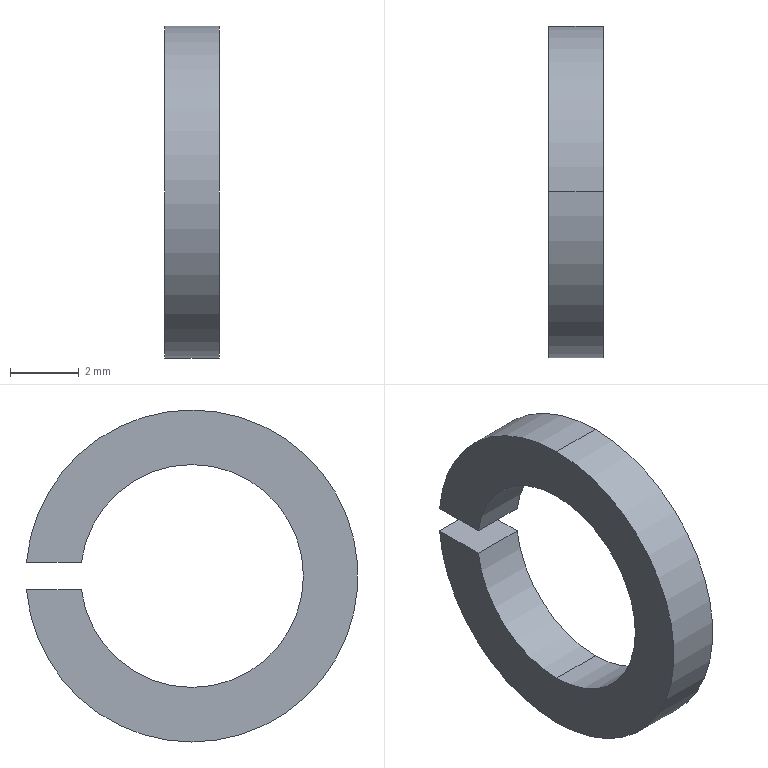Component | SolidWorks | GB_T93-1987StandardTypeSpringWasher(Assembly)6x1.6-1 | 1 solid | 10 faces | box 1.6 x 9.67 x 9.68 mm | volume 63 mm3 | cylinder 6 | plane 4 | commonest cylinder face diameters 6.5 x3 9.684 x3
build123d program:
from build123d import *

# Parameters (mm, degrees)
EXTRUDE1_DEPTH = 1.6


with BuildPart() as part:
    # Sketch1 → Extrude1 (new body)
    with BuildSketch(Plane.XY):
        with BuildLine():
            Line((-0.4, 4.825), (-0.4, 3.225))
            ThreePointArc((-0.4, 3.225), (0, -3.25), (0.4, 3.225))
            Line((0.4, 3.225), (0.4, 4.825))
            ThreePointArc((0.4, 4.825), (0, -4.842), (-0.4, 4.825))
        make_face()
    extrude(amount=EXTRUDE1_DEPTH)


solid = part.part

# Placed as in the assembly
solid = solid.moved(Location((-514.8, 30, 325), (0, 90, 0)))
STEP:
#1=CARTESIAN_POINT('',(-20.205,1.181,12.667));
#2=VERTEX_POINT('',#1);
#3=CARTESIAN_POINT('',(-20.205,1.181,12.923));
#4=VERTEX_POINT('',#3);
#5=CARTESIAN_POINT('',(-20.205,1.181,12.795));
#6=DIRECTION('',(-1.,0.,0.));
#7=DIRECTION('',(0.,0.,-1.));
#8=AXIS2_PLACEMENT_3D('',#5,#6,#7);
#9=CIRCLE('',#8,0.128);
#10=EDGE_CURVE('',#2,#4,#9,.T.);
#11=ORIENTED_EDGE('',*,*,#10,.F.);
#12=CARTESIAN_POINT('',(-20.268,1.181,12.667));
#13=VERTEX_POINT('',#12);
#14=CARTESIAN_POINT('',(-20.205,1.181,12.667));
#15=DIRECTION('',(-1.,0.,0.));
#16=VECTOR('',#15,39.37);
#17=LINE('',#14,#16);
#18=EDGE_CURVE('',#2,#13,#17,.T.);
#19=ORIENTED_EDGE('',*,*,#18,.T.);
#20=CARTESIAN_POINT('',(-20.268,1.181,12.923));
#21=VERTEX_POINT('',#20);
#22=CARTESIAN_POINT('',(-20.268,1.181,12.795));
#23=DIRECTION('',(-1.,0.,0.));
#24=DIRECTION('',(0.,0.,-1.));
#25=AXIS2_PLACEMENT_3D('',#22,#23,#24);
#26=CIRCLE('',#25,0.128);
#27=EDGE_CURVE('',#13,#21,#26,.T.);
#28=ORIENTED_EDGE('',*,*,#27,.T.);
#29=CARTESIAN_POINT('',(-20.205,1.181,12.923));
#30=DIRECTION('',(-1.,0.,0.));
#31=VECTOR('',#30,39.37);
#32=LINE('',#29,#31);
#33=EDGE_CURVE('',#4,#21,#32,.T.);
#34=ORIENTED_EDGE('',*,*,#33,.F.);
#35=EDGE_LOOP('',(#11,#19,#28,#34));
#36=FACE_OUTER_BOUND('',#35,.T.);
#37=CARTESIAN_POINT('',(-20.205,1.181,12.795));
#38=DIRECTION('',(-1.,0.,0.));
#39=DIRECTION('',(0.,0.,1.));
#40=AXIS2_PLACEMENT_3D('',#37,#38,#39);
#41=CYLINDRICAL_SURFACE('',#40,0.128);
#42=ADVANCED_FACE('',(#36),#41,.F.);
#43=CARTESIAN_POINT('',(-20.205,1.308,12.811));
#44=VERTEX_POINT('',#43);
#45=CARTESIAN_POINT('',(-20.205,1.181,12.795));
#46=DIRECTION('',(-1.,0.,0.));
#47=DIRECTION('',(0.,0.,-1.));
#48=AXIS2_PLACEMENT_3D('',#45,#46,#47);
#49=CIRCLE('',#48,0.128);
#50=EDGE_CURVE('',#4,#44,#49,.T.);
#51=ORIENTED_EDGE('',*,*,#50,.F.);
#52=ORIENTED_EDGE('',*,*,#33,.T.);
#53=CARTESIAN_POINT('',(-20.268,1.308,12.811));
#54=VERTEX_POINT('',#53);
#55=CARTESIAN_POINT('',(-20.268,1.181,12.795));
#56=DIRECTION('',(-1.,0.,0.));
#57=DIRECTION('',(0.,0.,-1.));
#58=AXIS2_PLACEMENT_3D('',#55,#56,#57);
#59=CIRCLE('',#58,0.128);
#60=EDGE_CURVE('',#21,#54,#59,.T.);
#61=ORIENTED_EDGE('',*,*,#60,.T.);
#62=CARTESIAN_POINT('',(-20.205,1.308,12.811));
#63=DIRECTION('',(-1.,0.,0.));
#64=VECTOR('',#63,39.37);
#65=LINE('',#62,#64);
#66=EDGE_CURVE('',#44,#54,#65,.T.);
#67=ORIENTED_EDGE('',*,*,#66,.F.);
#68=EDGE_LOOP('',(#51,#52,#61,#67));
#69=FACE_OUTER_BOUND('',#68,.T.);
#70=CARTESIAN_POINT('',(-20.205,1.181,12.795));
#71=DIRECTION('',(-1.,0.,0.));
#72=DIRECTION('',(0.,0.,1.));
#73=AXIS2_PLACEMENT_3D('',#70,#71,#72);
#74=CYLINDRICAL_SURFACE('',#73,0.128);
#75=ADVANCED_FACE('',(#69),#74,.F.);
#76=CARTESIAN_POINT('',(-20.205,1.181,12.605));
#77=VERTEX_POINT('',#76);
#78=CARTESIAN_POINT('',(-20.205,1.371,12.78));
#79=VERTEX_POINT('',#78);
#80=CARTESIAN_POINT('',(-20.205,1.181,12.795));
#81=DIRECTION('',(1.,0.,0.));
#82=DIRECTION('',(0.,0.,-1.));
#83=AXIS2_PLACEMENT_3D('',#80,#81,#82);
#84=CIRCLE('',#83,0.1906);
#85=EDGE_CURVE('',#77,#79,#84,.T.);
#86=ORIENTED_EDGE('',*,*,#85,.F.);
#87=CARTESIAN_POINT('',(-20.268,1.181,12.605));
#88=VERTEX_POINT('',#87);
#89=CARTESIAN_POINT('',(-20.205,1.181,12.605));
#90=DIRECTION('',(-1.,0.,0.));
#91=VECTOR('',#90,39.37);
#92=LINE('',#89,#91);
#93=EDGE_CURVE('',#77,#88,#92,.T.);
#94=ORIENTED_EDGE('',*,*,#93,.T.);
#95=CARTESIAN_POINT('',(-20.268,1.371,12.78));
#96=VERTEX_POINT('',#95);
#97=CARTESIAN_POINT('',(-20.268,1.181,12.795));
#98=DIRECTION('',(1.,0.,0.));
#99=DIRECTION('',(0.,0.,-1.));
#100=AXIS2_PLACEMENT_3D('',#97,#98,#99);
#101=CIRCLE('',#100,0.1906);
#102=EDGE_CURVE('',#88,#96,#101,.T.);
#103=ORIENTED_EDGE('',*,*,#102,.T.);
#104=CARTESIAN_POINT('',(-20.205,1.371,12.78));
#105=DIRECTION('',(-1.,0.,0.));
#106=VECTOR('',#105,39.37);
#107=LINE('',#104,#106);
#108=EDGE_CURVE('',#79,#96,#107,.T.);
#109=ORIENTED_EDGE('',*,*,#108,.F.);
#110=EDGE_LOOP('',(#86,#94,#103,#109));
#111=FACE_OUTER_BOUND('',#110,.T.);
#112=CARTESIAN_POINT('',(-20.205,1.181,12.795));
#113=DIRECTION('',(-1.,0.,0.));
#114=DIRECTION('',(0.,0.,1.));
#115=AXIS2_PLACEMENT_3D('',#112,#113,#114);
#116=CYLINDRICAL_SURFACE('',#115,0.1906);
#117=ADVANCED_FACE('',(#111),#116,.T.);
#118=ORIENTED_EDGE('',*,*,#93,.F.);
#119=CARTESIAN_POINT('',(-20.205,1.181,12.986));
#120=VERTEX_POINT('',#119);
#121=CARTESIAN_POINT('',(-20.205,1.181,12.795));
#122=DIRECTION('',(1.,0.,0.));
#123=DIRECTION('',(0.,0.,-1.));
#124=AXIS2_PLACEMENT_3D('',#121,#122,#123);
#125=CIRCLE('',#124,0.1906);
#126=EDGE_CURVE('',#120,#77,#125,.T.);
#127=ORIENTED_EDGE('',*,*,#126,.F.);
#128=CARTESIAN_POINT('',(-20.268,1.181,12.986));
#129=VERTEX_POINT('',#128);
#130=CARTESIAN_POINT('',(-20.205,1.181,12.986));
#131=DIRECTION('',(-1.,0.,0.));
#132=VECTOR('',#131,39.37);
#133=LINE('',#130,#132);
#134=EDGE_CURVE('',#120,#129,#133,.T.);
#135=ORIENTED_EDGE('',*,*,#134,.T.);
#136=CARTESIAN_POINT('',(-20.268,1.181,12.795));
#137=DIRECTION('',(1.,0.,0.));
#138=DIRECTION('',(0.,0.,-1.));
#139=AXIS2_PLACEMENT_3D('',#136,#137,#138);
#140=CIRCLE('',#139,0.1906);
#141=EDGE_CURVE('',#129,#88,#140,.T.);
#142=ORIENTED_EDGE('',*,*,#141,.T.);
#143=EDGE_LOOP('',(#118,#127,#135,#142));
#144=FACE_OUTER_BOUND('',#143,.T.);
#145=CARTESIAN_POINT('',(-20.205,1.181,12.795));
#146=DIRECTION('',(-1.,0.,0.));
#147=DIRECTION('',(0.,0.,1.));
#148=AXIS2_PLACEMENT_3D('',#145,#146,#147);
#149=CYLINDRICAL_SURFACE('',#148,0.1906);
#150=ADVANCED_FACE('',(#144),#149,.T.);
#151=ORIENTED_EDGE('',*,*,#134,.F.);
#152=CARTESIAN_POINT('',(-20.205,1.371,12.811));
#153=VERTEX_POINT('',#152);
#154=CARTESIAN_POINT('',(-20.205,1.181,12.795));
#155=DIRECTION('',(1.,0.,0.));
#156=DIRECTION('',(0.,0.,-1.));
#157=AXIS2_PLACEMENT_3D('',#154,#155,#156);
#158=CIRCLE('',#157,0.1906);
#159=EDGE_CURVE('',#153,#120,#158,.T.);
#160=ORIENTED_EDGE('',*,*,#159,.F.);
#161=CARTESIAN_POINT('',(-20.268,1.371,12.811));
#162=VERTEX_POINT('',#161);
#163=CARTESIAN_POINT('',(-20.205,1.371,12.811));
#164=DIRECTION('',(-1.,0.,0.));
#165=VECTOR('',#164,39.37);
#166=LINE('',#163,#165);
#167=EDGE_CURVE('',#153,#162,#166,.T.);
#168=ORIENTED_EDGE('',*,*,#167,.T.);
#169=CARTESIAN_POINT('',(-20.268,1.181,12.795));
#170=DIRECTION('',(1.,0.,0.));
#171=DIRECTION('',(0.,0.,-1.));
#172=AXIS2_PLACEMENT_3D('',#169,#170,#171);
#173=CIRCLE('',#172,0.1906);
#174=EDGE_CURVE('',#162,#129,#173,.T.);
#175=ORIENTED_EDGE('',*,*,#174,.T.);
#176=EDGE_LOOP('',(#151,#160,#168,#175));
#177=FACE_OUTER_BOUND('',#176,.T.);
#178=CARTESIAN_POINT('',(-20.205,1.181,12.795));
#179=DIRECTION('',(-1.,0.,0.));
#180=DIRECTION('',(0.,0.,1.));
#181=AXIS2_PLACEMENT_3D('',#178,#179,#180);
#182=CYLINDRICAL_SURFACE('',#181,0.1906);
#183=ADVANCED_FACE('',(#177),#182,.T.);
#184=CARTESIAN_POINT('',(-20.268,1.308,12.78));
#185=VERTEX_POINT('',#184);
#186=CARTESIAN_POINT('',(-20.268,1.371,12.78));
#187=DIRECTION('',(0.,-1.,-0.));
#188=VECTOR('',#187,39.37);
#189=LINE('',#186,#188);
#190=EDGE_CURVE('',#96,#185,#189,.T.);
#191=ORIENTED_EDGE('',*,*,#190,.T.);
#192=CARTESIAN_POINT('',(-20.205,1.308,12.78));
#193=VERTEX_POINT('',#192);
#194=CARTESIAN_POINT('',(-20.205,1.308,12.78));
#195=DIRECTION('',(-1.,0.,0.));
#196=VECTOR('',#195,39.37);
#197=LINE('',#194,#196);
#198=EDGE_CURVE('',#193,#185,#197,.T.);
#199=ORIENTED_EDGE('',*,*,#198,.F.);
#200=CARTESIAN_POINT('',(-20.205,1.371,12.78));
#201=DIRECTION('',(0.,-1.,-0.));
#202=VECTOR('',#201,39.37);
#203=LINE('',#200,#202);
#204=EDGE_CURVE('',#79,#193,#203,.T.);
#205=ORIENTED_EDGE('',*,*,#204,.F.);
#206=ORIENTED_EDGE('',*,*,#108,.T.);
#207=EDGE_LOOP('',(#191,#199,#205,#206));
#208=FACE_OUTER_BOUND('',#207,.T.);
#209=CARTESIAN_POINT('',(-20.205,1.371,12.78));
#210=DIRECTION('',(0.,0.,-1.));
#211=DIRECTION('',(0.,1.,0.));
#212=AXIS2_PLACEMENT_3D('',#209,#210,#211);
#213=PLANE('',#212);
#214=ADVANCED_FACE('',(#208),#213,.F.);
#215=ORIENTED_EDGE('',*,*,#18,.F.);
#216=CARTESIAN_POINT('',(-20.205,1.181,12.795));
#217=DIRECTION('',(-1.,0.,0.));
#218=DIRECTION('',(0.,0.,-1.));
#219=AXIS2_PLACEMENT_3D('',#216,#217,#218);
#220=CIRCLE('',#219,0.128);
#221=EDGE_CURVE('',#193,#2,#220,.T.);
#222=ORIENTED_EDGE('',*,*,#221,.F.);
#223=ORIENTED_EDGE('',*,*,#198,.T.);
#224=CARTESIAN_POINT('',(-20.268,1.181,12.795));
#225=DIRECTION('',(-1.,0.,0.));
#226=DIRECTION('',(0.,0.,-1.));
#227=AXIS2_PLACEMENT_3D('',#224,#225,#226);
#228=CIRCLE('',#227,0.128);
#229=EDGE_CURVE('',#185,#13,#228,.T.);
#230=ORIENTED_EDGE('',*,*,#229,.T.);
#231=EDGE_LOOP('',(#215,#222,#223,#230));
#232=FACE_OUTER_BOUND('',#231,.T.);
#233=CARTESIAN_POINT('',(-20.205,1.181,12.795));
#234=DIRECTION('',(-1.,0.,0.));
#235=DIRECTION('',(0.,0.,1.));
#236=AXIS2_PLACEMENT_3D('',#233,#234,#235);
#237=CYLINDRICAL_SURFACE('',#236,0.128);
#238=ADVANCED_FACE('',(#232),#237,.F.);
#239=CARTESIAN_POINT('',(-20.268,1.371,12.811));
#240=DIRECTION('',(0.,1.,0.));
#241=VECTOR('',#240,39.37);
#242=LINE('',#239,#241);
#243=EDGE_CURVE('',#54,#162,#242,.T.);
#244=ORIENTED_EDGE('',*,*,#243,.T.);
#245=ORIENTED_EDGE('',*,*,#167,.F.);
#246=CARTESIAN_POINT('',(-20.205,1.371,12.811));
#247=DIRECTION('',(0.,1.,0.));
#248=VECTOR('',#247,39.37);
#249=LINE('',#246,#248);
#250=EDGE_CURVE('',#44,#153,#249,.T.);
#251=ORIENTED_EDGE('',*,*,#250,.F.);
#252=ORIENTED_EDGE('',*,*,#66,.T.);
#253=EDGE_LOOP('',(#244,#245,#251,#252));
#254=FACE_OUTER_BOUND('',#253,.T.);
#255=CARTESIAN_POINT('',(-20.205,1.371,12.811));
#256=DIRECTION('',(0.,-0.,1.));
#257=DIRECTION('',(0.,-1.,-0.));
#258=AXIS2_PLACEMENT_3D('',#255,#256,#257);
#259=PLANE('',#258);
#260=ADVANCED_FACE('',(#254),#259,.F.);
#261=ORIENTED_EDGE('',*,*,#159,.T.);
#262=ORIENTED_EDGE('',*,*,#126,.T.);
#263=ORIENTED_EDGE('',*,*,#85,.T.);
#264=ORIENTED_EDGE('',*,*,#204,.T.);
#265=ORIENTED_EDGE('',*,*,#221,.T.);
#266=ORIENTED_EDGE('',*,*,#10,.T.);
#267=ORIENTED_EDGE('',*,*,#50,.T.);
#268=ORIENTED_EDGE('',*,*,#250,.T.);
#269=EDGE_LOOP('',(#261,#262,#263,#264,#265,#266,#267,#268));
#270=FACE_OUTER_BOUND('',#269,.T.);
#271=CARTESIAN_POINT('',(-20.205,1.181,12.795));
#272=DIRECTION('',(1.,0.,0.));
#273=DIRECTION('',(0.,0.,-1.));
#274=AXIS2_PLACEMENT_3D('',#271,#272,#273);
#275=PLANE('',#274);
#276=ADVANCED_FACE('',(#270),#275,.T.);
#277=ORIENTED_EDGE('',*,*,#174,.F.);
#278=ORIENTED_EDGE('',*,*,#243,.F.);
#279=ORIENTED_EDGE('',*,*,#60,.F.);
#280=ORIENTED_EDGE('',*,*,#27,.F.);
#281=ORIENTED_EDGE('',*,*,#229,.F.);
#282=ORIENTED_EDGE('',*,*,#190,.F.);
#283=ORIENTED_EDGE('',*,*,#102,.F.);
#284=ORIENTED_EDGE('',*,*,#141,.F.);
#285=EDGE_LOOP('',(#277,#278,#279,#280,#281,#282,#283,#284));
#286=FACE_OUTER_BOUND('',#285,.T.);
#287=CARTESIAN_POINT('',(-20.268,1.181,12.795));
#288=DIRECTION('',(1.,0.,0.));
#289=DIRECTION('',(0.,0.,-1.));
#290=AXIS2_PLACEMENT_3D('',#287,#288,#289);
#291=PLANE('',#290);
#292=ADVANCED_FACE('',(#286),#291,.F.);
#293=CLOSED_SHELL('',(#42,#75,#117,#150,#183,#214,#238,#260,#276,#292));
#294=MANIFOLD_SOLID_BREP('',#293);
#295=CARTESIAN_POINT('',(0.,0.,0.));
#296=DIRECTION('',(0.,0.,1.));
#297=DIRECTION('',(1.,0.,0.));
#298=AXIS2_PLACEMENT_3D('',#295,#296,#297);
#299=(LENGTH_UNIT()NAMED_UNIT(*)SI_UNIT($,.METRE.));
#300=LENGTH_MEASURE_WITH_UNIT(LENGTH_MEASURE(0.0254),#299);
#301=DIMENSIONAL_EXPONENTS(1.,0.,0.,0.,0.,0.,0.);
#302=(CONVERSION_BASED_UNIT('',#300)LENGTH_UNIT()NAMED_UNIT(#301));
#303=UNCERTAINTY_MEASURE_WITH_UNIT(LENGTH_MEASURE(0.00001),#302,'','');
#304=(NAMED_UNIT(*)PLANE_ANGLE_UNIT()SI_UNIT($,.RADIAN.));
#305=(NAMED_UNIT(*)SI_UNIT($,.STERADIAN.)SOLID_ANGLE_UNIT());
#306=(GEOMETRIC_REPRESENTATION_CONTEXT(3)GLOBAL_UNCERTAINTY_ASSIGNED_CONTEXT((#303))GLOBAL_UNIT_ASSIGNED_CONTEXT((#302,#304,#305))REPRESENTATION_CONTEXT('',''));
#307=ADVANCED_BREP_SHAPE_REPRESENTATION('',(#294,#298),#306);
#308=COLOUR_RGB('',0.7922,0.8196,0.9333);
#309=FILL_AREA_STYLE_COLOUR('',#308);
#310=FILL_AREA_STYLE('',(#309));
#311=SURFACE_STYLE_FILL_AREA(#310);
#312=SURFACE_SIDE_STYLE('',(#311));
#313=SURFACE_STYLE_USAGE(.BOTH.,#312);
#314=PRESENTATION_STYLE_ASSIGNMENT((#313));
#315=STYLED_ITEM('',(#314),#294);
#316=PRESENTATION_LAYER_ASSIGNMENT('','',(#315));
#317=(LENGTH_UNIT()NAMED_UNIT(*)SI_UNIT($,.METRE.));
#318=LENGTH_MEASURE_WITH_UNIT(LENGTH_MEASURE(0.0254),#317);
#319=DIMENSIONAL_EXPONENTS(1.,0.,0.,0.,0.,0.,0.);
#320=(CONVERSION_BASED_UNIT('',#318)LENGTH_UNIT()NAMED_UNIT(#319));
#321=UNCERTAINTY_MEASURE_WITH_UNIT(LENGTH_MEASURE(0.00001),#320,'','');
#322=(NAMED_UNIT(*)PLANE_ANGLE_UNIT()SI_UNIT($,.RADIAN.));
#323=(NAMED_UNIT(*)SI_UNIT($,.STERADIAN.)SOLID_ANGLE_UNIT());
#324=(GEOMETRIC_REPRESENTATION_CONTEXT(3)GLOBAL_UNCERTAINTY_ASSIGNED_CONTEXT((#321))GLOBAL_UNIT_ASSIGNED_CONTEXT((#320,#322,#323))REPRESENTATION_CONTEXT('',''));
#325=MECHANICAL_DESIGN_GEOMETRIC_PRESENTATION_REPRESENTATION('',(#315),#324);